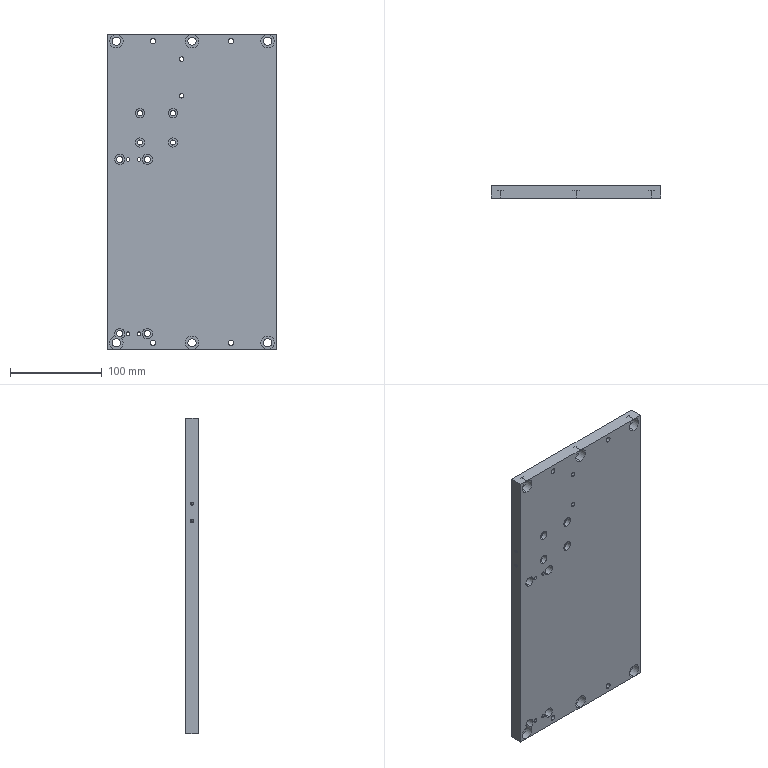Component | SolidWorks | FlipMechanismA-17-1 | 1 solid | 124 faces | box 185 x 14 x 344 mm | volume 868807 mm3 | cylinder 89 | plane 27 | cone 8 | commonest cylinder face diameters 6 x14 9 x12 14.8 x11 10 x8 4 x8 11 x8 6.6 x8 3.3 x8
build123d program:
from build123d import *

# Parameters (mm, degrees)
SKETCH1_W                                       = 185
SKETCH1_H                                       = 344
EXTRUDE1_DEPTH                                  = 7
M8_HEX_SOCKET_HEAD_CAP_SCREW_CBORE2_D           = 9
M8_HEX_SOCKET_HEAD_CAP_SCREW_CBORE2_CBORE_D     = 14.8
M8_HEX_SOCKET_HEAD_CAP_SCREW_CBORE2_CBORE_DEPTH = 8.6
SKETCH3_R                                       = 3
CUT_EXTRUDE1_DEPTH                              = 83
SKETCH13_R                                      = 3
CUT_EXTRUDE3_DEPTH                              = 8
M4_TAPPED_HOLE1_D                               = 3.3
M4_TAPPED_HOLE1_DEPTH                           = 11.5
M4_TAPPED_HOLE1_TIP                             = 0.9914
M6_TAPPED_HOLE1_D                               = 5
M6_TAPPED_HOLE1_DEPTH                           = 17
M6_TAPPED_HOLE1_TIP                             = 1.502
M4_TAPPED_HOLE2_D                               = 3.3
M4_TAPPED_HOLE2_DEPTH                           = 10.1
M4_TAPPED_HOLE2_TIP                             = 0.9914
M6_HEX_SOCKET_HEAD_CAP_SCREW_CBORE2_D           = 6.6
M6_HEX_SOCKET_HEAD_CAP_SCREW_CBORE2_CBORE_D     = 11
M6_HEX_SOCKET_HEAD_CAP_SCREW_CBORE2_CBORE_DEPTH = 8.6
SKETCH22_R                                      = 2
CUT_EXTRUDE4_DEPTH                              = 32
M5_HEX_SOCKET_HEAD_CAP_SCREW_CBORE2_D           = 5.5
M5_HEX_SOCKET_HEAD_CAP_SCREW_CBORE2_CBORE_D     = 10
M5_HEX_SOCKET_HEAD_CAP_SCREW_CBORE2_CBORE_DEPTH = 5.4
SKETCH2_W                                       = 51.5
SKETCH2_H                                       = 45
GUIDEBLOCKSEATPOCKET_DEPTH                      = 0.4


with BuildPart() as part:
    # Sketch1 → Extrude1 (new, symmetric)
    with BuildSketch(Plane(origin=(0, 0, 0), x_dir=(1, 0, 0), z_dir=(0, 1, 0))):
        Rectangle(SKETCH1_W, SKETCH1_H)
    extrude(amount=EXTRUDE1_DEPTH, both=True)

    # M8 Hex Socket Head Cap Screw CBORE2 (through all)
    with Locations(Plane(origin=(0, -7, 0), x_dir=(-1, 0, 0), z_dir=(0, -1, 0))):
        with Locations((82.5, 164.5), (0, 164.5), (-82.5, 164.5), (82.5, -164.5), (0, -164.5), (-82.5, -164.5)):
            CounterBoreHole(M8_HEX_SOCKET_HEAD_CAP_SCREW_CBORE2_D / 2, M8_HEX_SOCKET_HEAD_CAP_SCREW_CBORE2_CBORE_D / 2, M8_HEX_SOCKET_HEAD_CAP_SCREW_CBORE2_CBORE_DEPTH)

    # Sketch3 → Cut-Extrude1 (cut)
    with BuildSketch(Plane.XZ.offset(7)):
        with Locations(Location((-42.5, -164.5, 0), (0, 0, 270))):
            Circle(SKETCH3_R)
        with Locations(Location((42.5, -164.5, 0), (0, 0, 270))):
            Circle(SKETCH3_R)
        with Locations(Location((42.5, 164.5, 0), (0, 0, 90))):
            Circle(SKETCH3_R)
        with Locations(Location((-42.5, 164.5, 0), (0, 0, 90))):
            Circle(SKETCH3_R)
    extrude(amount=-CUT_EXTRUDE1_DEPTH, mode=Mode.SUBTRACT)

    # Sketch13 → Cut-Extrude3 (cut)
    with BuildSketch(Plane(origin=(0, 7, 0), x_dir=(1, 0, 0), z_dir=(0, 1, 0))):
        with Locations(Location((69.5, 95, 0), (0, 0, 270))):
            Circle(SKETCH13_R)
        with Locations(Location((9.5, 95, 0), (0, 0, 270))):
            Circle(SKETCH13_R)
        with Locations(Location((80.5, 70, 0), (0, 0, 270))):
            Circle(SKETCH13_R)
    extrude(amount=-CUT_EXTRUDE3_DEPTH, mode=Mode.SUBTRACT)

    # M4 Tapped Hole1
    with Locations(Plane.ZY.offset(92.5)):
        with Locations((-79.5, 0), (-60.5, 0)):
            Hole(M4_TAPPED_HOLE1_D / 2, depth=M4_TAPPED_HOLE1_DEPTH)
            with Locations((0, 0, -(M4_TAPPED_HOLE1_DEPTH + M4_TAPPED_HOLE1_TIP / 2))):  # 118° drill point
                Cone(0, M4_TAPPED_HOLE1_D / 2, M4_TAPPED_HOLE1_TIP, mode=Mode.SUBTRACT)

    # M6 Tapped Hole1
    with Locations(Plane(origin=(0, 7, 0), x_dir=(1, 0, 0), z_dir=(0, 1, 0))):
        with Locations((11.25, 145), (11.25, 105)):
            Hole(M6_TAPPED_HOLE1_D / 2, depth=M6_TAPPED_HOLE1_DEPTH)
            with Locations((0, 0, -(M6_TAPPED_HOLE1_DEPTH + M6_TAPPED_HOLE1_TIP / 2))):  # 118° drill point
                Cone(0, M6_TAPPED_HOLE1_D / 2, M6_TAPPED_HOLE1_TIP, mode=Mode.SUBTRACT)

    # M4 Tapped Hole2
    with Locations(Plane(origin=(92.5, 0, 0), x_dir=(0, 0, -1), z_dir=(1, 0, 0))):
        with Locations((60, 0), (79, 0)):
            Hole(M4_TAPPED_HOLE2_D / 2, depth=M4_TAPPED_HOLE2_DEPTH)
            with Locations((0, 0, -(M4_TAPPED_HOLE2_DEPTH + M4_TAPPED_HOLE2_TIP / 2))):  # 118° drill point
                Cone(0, M4_TAPPED_HOLE2_D / 2, M4_TAPPED_HOLE2_TIP, mode=Mode.SUBTRACT)

    # M6 Hex Socket Head Cap Screw CBORE2 (through all)
    with Locations(Plane(origin=(0, -7, 0), x_dir=(-1, 0, 0), z_dir=(0, -1, 0))):
        with Locations((-48.75, 35.5), (-78.75, 35.5), (-48.75, -154.5), (-78.75, -154.5)):
            CounterBoreHole(M6_HEX_SOCKET_HEAD_CAP_SCREW_CBORE2_D / 2, M6_HEX_SOCKET_HEAD_CAP_SCREW_CBORE2_CBORE_D / 2, M6_HEX_SOCKET_HEAD_CAP_SCREW_CBORE2_CBORE_DEPTH)

    # Sketch22 → Cut-Extrude4 (cut)
    with BuildSketch(Plane.XZ.offset(7)):
        with Locations(Location((57.75, -35.5, 0), (0, 0, 270))):
            Circle(SKETCH22_R)
        with Locations(Location((69.75, -35.5, 0), (0, 0, 270))):
            Circle(SKETCH22_R)
        with Locations(Location((57.75, 154.5, 0), (0, 0, 270))):
            Circle(SKETCH22_R)
        with Locations(Location((69.75, 154.5, 0), (0, 0, 270))):
            Circle(SKETCH22_R)
    extrude(amount=-CUT_EXTRUDE4_DEPTH, mode=Mode.SUBTRACT)

    # M5 Hex Socket Head Cap Screw CBORE2 (through all)
    with Locations(Plane(origin=(0, -7, 0), x_dir=(-1, 0, 0), z_dir=(0, -1, 0))):
        with Locations((-20.75, 86), (-20.75, 54), (-56.75, 54), (-56.75, 86)):
            CounterBoreHole(M5_HEX_SOCKET_HEAD_CAP_SCREW_CBORE2_D / 2, M5_HEX_SOCKET_HEAD_CAP_SCREW_CBORE2_CBORE_D / 2, M5_HEX_SOCKET_HEAD_CAP_SCREW_CBORE2_CBORE_DEPTH)

    # Sketch2 → GuideBlockSeatPocket (cut)
    with BuildSketch(Plane(origin=(0, 7, 0), x_dir=(1, 0, 0), z_dir=(0, 1, 0))):
        with Locations((38.75, 70)):
            Rectangle(SKETCH2_W, SKETCH2_H)
    extrude(amount=-GUIDEBLOCKSEATPOCKET_DEPTH, mode=Mode.SUBTRACT)


solid = part.part

# Placed as in the assembly
solid = solid.moved(Location((-22.5, -46.6, -125), (-180, 0, 180)))